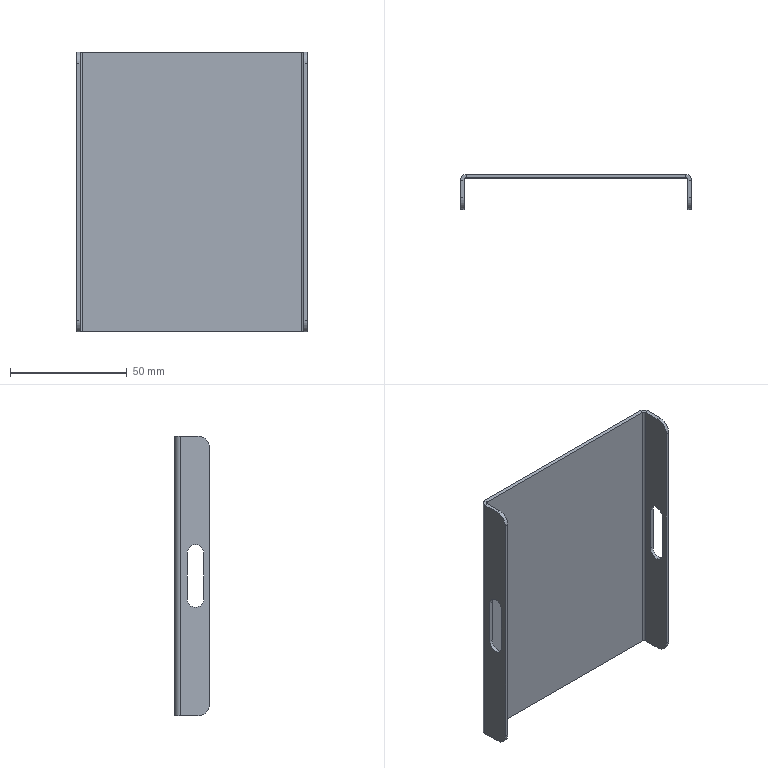Component | SolidWorks | AA-1_CoverPlate-1 | 1 solid | 36 faces | box 99 x 15 x 120 mm | volume 21842 mm3 | plane 22 | cylinder 14 | commonest cylinder face diameters 7 x6 10 x4 5 x2 2 x2
STEP:
#1=CARTESIAN_POINT('',(-19.184,-10.286,29.016));
#2=VERTEX_POINT('',#1);
#3=CARTESIAN_POINT('',(-19.184,-10.148,28.878));
#4=VERTEX_POINT('',#3);
#5=CARTESIAN_POINT('',(-19.184,-10.286,28.878));
#6=DIRECTION('',(-1.,0.,-0.));
#7=DIRECTION('',(0.,-1.,0.));
#8=AXIS2_PLACEMENT_3D('',#5,#6,#7);
#9=CIRCLE('',#8,0.1378);
#10=EDGE_CURVE('',#2,#4,#9,.T.);
#11=ORIENTED_EDGE('',*,*,#10,.F.);
#12=CARTESIAN_POINT('',(-19.243,-10.286,29.016));
#13=VERTEX_POINT('',#12);
#14=CARTESIAN_POINT('',(-15.345,-10.286,29.016));
#15=DIRECTION('',(-1.,0.,-0.));
#16=VECTOR('',#15,39.37);
#17=LINE('',#14,#16);
#18=EDGE_CURVE('',#2,#13,#17,.T.);
#19=ORIENTED_EDGE('',*,*,#18,.T.);
#20=CARTESIAN_POINT('',(-19.243,-10.148,28.878));
#21=VERTEX_POINT('',#20);
#22=CARTESIAN_POINT('',(-19.243,-10.286,28.878));
#23=DIRECTION('',(-1.,0.,-0.));
#24=DIRECTION('',(0.,0.,1.));
#25=AXIS2_PLACEMENT_3D('',#22,#23,#24);
#26=CIRCLE('',#25,0.1378);
#27=EDGE_CURVE('',#13,#21,#26,.T.);
#28=ORIENTED_EDGE('',*,*,#27,.T.);
#29=CARTESIAN_POINT('',(-15.345,-10.148,28.878));
#30=DIRECTION('',(-1.,0.,-0.));
#31=VECTOR('',#30,39.37);
#32=LINE('',#29,#31);
#33=EDGE_CURVE('',#4,#21,#32,.T.);
#34=ORIENTED_EDGE('',*,*,#33,.F.);
#35=EDGE_LOOP('',(#11,#19,#28,#34));
#36=FACE_OUTER_BOUND('',#35,.T.);
#37=CARTESIAN_POINT('',(-15.345,-10.286,28.878));
#38=DIRECTION('',(-1.,0.,-0.));
#39=DIRECTION('',(0.,0.,1.));
#40=AXIS2_PLACEMENT_3D('',#37,#38,#39);
#41=CYLINDRICAL_SURFACE('',#40,0.1378);
#42=ADVANCED_FACE('',(#36),#41,.F.);
#43=CARTESIAN_POINT('',(-15.345,-10.286,29.016));
#44=VERTEX_POINT('',#43);
#45=CARTESIAN_POINT('',(-15.345,-10.148,28.878));
#46=VERTEX_POINT('',#45);
#47=CARTESIAN_POINT('',(-15.345,-10.286,28.878));
#48=DIRECTION('',(-1.,0.,-0.));
#49=DIRECTION('',(0.,0.,1.));
#50=AXIS2_PLACEMENT_3D('',#47,#48,#49);
#51=CIRCLE('',#50,0.1378);
#52=EDGE_CURVE('',#44,#46,#51,.T.);
#53=ORIENTED_EDGE('',*,*,#52,.F.);
#54=CARTESIAN_POINT('',(-15.404,-10.286,29.016));
#55=VERTEX_POINT('',#54);
#56=CARTESIAN_POINT('',(-15.345,-10.286,29.016));
#57=DIRECTION('',(-1.,0.,-0.));
#58=VECTOR('',#57,39.37);
#59=LINE('',#56,#58);
#60=EDGE_CURVE('',#44,#55,#59,.T.);
#61=ORIENTED_EDGE('',*,*,#60,.T.);
#62=CARTESIAN_POINT('',(-15.404,-10.148,28.878));
#63=VERTEX_POINT('',#62);
#64=CARTESIAN_POINT('',(-15.404,-10.286,28.878));
#65=DIRECTION('',(-1.,-0.,-0.));
#66=DIRECTION('',(0.,-1.,0.));
#67=AXIS2_PLACEMENT_3D('',#64,#65,#66);
#68=CIRCLE('',#67,0.1378);
#69=EDGE_CURVE('',#55,#63,#68,.T.);
#70=ORIENTED_EDGE('',*,*,#69,.T.);
#71=CARTESIAN_POINT('',(-15.345,-10.148,28.878));
#72=DIRECTION('',(-1.,0.,-0.));
#73=VECTOR('',#72,39.37);
#74=LINE('',#71,#73);
#75=EDGE_CURVE('',#46,#63,#74,.T.);
#76=ORIENTED_EDGE('',*,*,#75,.F.);
#77=EDGE_LOOP('',(#53,#61,#70,#76));
#78=FACE_OUTER_BOUND('',#77,.T.);
#79=CARTESIAN_POINT('',(-15.345,-10.286,28.878));
#80=DIRECTION('',(-1.,0.,-0.));
#81=DIRECTION('',(0.,0.,1.));
#82=AXIS2_PLACEMENT_3D('',#79,#80,#81);
#83=CYLINDRICAL_SURFACE('',#82,0.1378);
#84=ADVANCED_FACE('',(#78),#83,.F.);
#85=CARTESIAN_POINT('',(-19.145,-9.932,30.846));
#86=VERTEX_POINT('',#85);
#87=CARTESIAN_POINT('',(-15.444,-9.932,30.846));
#88=VERTEX_POINT('',#87);
#89=CARTESIAN_POINT('',(-15.444,-9.932,30.846));
#90=DIRECTION('',(1.,-0.,0.));
#91=VECTOR('',#90,39.37);
#92=LINE('',#89,#91);
#93=EDGE_CURVE('',#86,#88,#92,.T.);
#94=ORIENTED_EDGE('',*,*,#93,.F.);
#95=CARTESIAN_POINT('',(-19.145,-9.991,30.846));
#96=VERTEX_POINT('',#95);
#97=CARTESIAN_POINT('',(-19.145,-9.991,30.846));
#98=DIRECTION('',(0.,1.,-0.));
#99=VECTOR('',#98,39.37);
#100=LINE('',#97,#99);
#101=EDGE_CURVE('',#96,#86,#100,.T.);
#102=ORIENTED_EDGE('',*,*,#101,.F.);
#103=CARTESIAN_POINT('',(-15.444,-9.991,30.846));
#104=VERTEX_POINT('',#103);
#105=CARTESIAN_POINT('',(-15.444,-9.991,30.846));
#106=DIRECTION('',(1.,-0.,0.));
#107=VECTOR('',#106,39.37);
#108=LINE('',#105,#107);
#109=EDGE_CURVE('',#96,#104,#108,.T.);
#110=ORIENTED_EDGE('',*,*,#109,.T.);
#111=CARTESIAN_POINT('',(-15.444,-9.991,30.846));
#112=DIRECTION('',(0.,1.,-0.));
#113=VECTOR('',#112,39.37);
#114=LINE('',#111,#113);
#115=EDGE_CURVE('',#104,#88,#114,.T.);
#116=ORIENTED_EDGE('',*,*,#115,.T.);
#117=EDGE_LOOP('',(#94,#102,#110,#116));
#118=FACE_OUTER_BOUND('',#117,.T.);
#119=CARTESIAN_POINT('',(-15.444,-9.991,30.846));
#120=DIRECTION('',(-0.,0.,1.));
#121=DIRECTION('',(1.,-0.,0.));
#122=AXIS2_PLACEMENT_3D('',#119,#120,#121);
#123=PLANE('',#122);
#124=ADVANCED_FACE('',(#118),#123,.T.);
#125=CARTESIAN_POINT('',(-15.444,-9.932,26.122));
#126=VERTEX_POINT('',#125);
#127=CARTESIAN_POINT('',(-19.145,-9.932,26.122));
#128=VERTEX_POINT('',#127);
#129=CARTESIAN_POINT('',(-15.444,-9.932,26.122));
#130=DIRECTION('',(-1.,0.,-0.));
#131=VECTOR('',#130,39.37);
#132=LINE('',#129,#131);
#133=EDGE_CURVE('',#126,#128,#132,.T.);
#134=ORIENTED_EDGE('',*,*,#133,.F.);
#135=CARTESIAN_POINT('',(-15.444,-9.991,26.122));
#136=VERTEX_POINT('',#135);
#137=CARTESIAN_POINT('',(-15.444,-9.991,26.122));
#138=DIRECTION('',(0.,1.,-0.));
#139=VECTOR('',#138,39.37);
#140=LINE('',#137,#139);
#141=EDGE_CURVE('',#136,#126,#140,.T.);
#142=ORIENTED_EDGE('',*,*,#141,.F.);
#143=CARTESIAN_POINT('',(-19.145,-9.991,26.122));
#144=VERTEX_POINT('',#143);
#145=CARTESIAN_POINT('',(-15.444,-9.991,26.122));
#146=DIRECTION('',(-1.,0.,-0.));
#147=VECTOR('',#146,39.37);
#148=LINE('',#145,#147);
#149=EDGE_CURVE('',#136,#144,#148,.T.);
#150=ORIENTED_EDGE('',*,*,#149,.T.);
#151=CARTESIAN_POINT('',(-19.145,-9.991,26.122));
#152=DIRECTION('',(0.,1.,-0.));
#153=VECTOR('',#152,39.37);
#154=LINE('',#151,#153);
#155=EDGE_CURVE('',#144,#128,#154,.T.);
#156=ORIENTED_EDGE('',*,*,#155,.T.);
#157=EDGE_LOOP('',(#134,#142,#150,#156));
#158=FACE_OUTER_BOUND('',#157,.T.);
#159=CARTESIAN_POINT('',(-15.444,-9.991,26.122));
#160=DIRECTION('',(0.,-0.,-1.));
#161=DIRECTION('',(-1.,0.,-0.));
#162=AXIS2_PLACEMENT_3D('',#159,#160,#161);
#163=PLANE('',#162);
#164=ADVANCED_FACE('',(#158),#163,.T.);
#165=ORIENTED_EDGE('',*,*,#109,.F.);
#166=CARTESIAN_POINT('',(-19.145,-9.991,26.122));
#167=DIRECTION('',(-0.,0.,1.));
#168=VECTOR('',#167,39.37);
#169=LINE('',#166,#168);
#170=EDGE_CURVE('',#144,#96,#169,.T.);
#171=ORIENTED_EDGE('',*,*,#170,.F.);
#172=ORIENTED_EDGE('',*,*,#149,.F.);
#173=CARTESIAN_POINT('',(-15.444,-9.991,26.122));
#174=DIRECTION('',(0.,-0.,-1.));
#175=VECTOR('',#174,39.37);
#176=LINE('',#173,#175);
#177=EDGE_CURVE('',#104,#136,#176,.T.);
#178=ORIENTED_EDGE('',*,*,#177,.F.);
#179=EDGE_LOOP('',(#165,#171,#172,#178));
#180=FACE_OUTER_BOUND('',#179,.T.);
#181=CARTESIAN_POINT('',(-17.294,-9.991,28.484));
#182=DIRECTION('',(0.,1.,-0.));
#183=DIRECTION('',(-1.,0.,-0.));
#184=AXIS2_PLACEMENT_3D('',#181,#182,#183);
#185=PLANE('',#184);
#186=ADVANCED_FACE('',(#180),#185,.F.);
#187=ORIENTED_EDGE('',*,*,#93,.T.);
#188=CARTESIAN_POINT('',(-15.444,-9.932,26.122));
#189=DIRECTION('',(0.,-0.,-1.));
#190=VECTOR('',#189,39.37);
#191=LINE('',#188,#190);
#192=EDGE_CURVE('',#88,#126,#191,.T.);
#193=ORIENTED_EDGE('',*,*,#192,.T.);
#194=ORIENTED_EDGE('',*,*,#133,.T.);
#195=CARTESIAN_POINT('',(-19.145,-9.932,26.122));
#196=DIRECTION('',(-0.,0.,1.));
#197=VECTOR('',#196,39.37);
#198=LINE('',#195,#197);
#199=EDGE_CURVE('',#128,#86,#198,.T.);
#200=ORIENTED_EDGE('',*,*,#199,.T.);
#201=EDGE_LOOP('',(#187,#193,#194,#200));
#202=FACE_OUTER_BOUND('',#201,.T.);
#203=CARTESIAN_POINT('',(-17.294,-9.932,28.484));
#204=DIRECTION('',(0.,1.,-0.));
#205=DIRECTION('',(-1.,0.,-0.));
#206=AXIS2_PLACEMENT_3D('',#203,#204,#205);
#207=PLANE('',#206);
#208=ADVANCED_FACE('',(#202),#207,.T.);
#209=CARTESIAN_POINT('',(-19.184,-10.03,30.846));
#210=VERTEX_POINT('',#209);
#211=CARTESIAN_POINT('',(-19.243,-10.03,30.846));
#212=VERTEX_POINT('',#211);
#213=CARTESIAN_POINT('',(-19.243,-10.03,30.846));
#214=DIRECTION('',(-1.,0.,-0.));
#215=VECTOR('',#214,39.37);
#216=LINE('',#213,#215);
#217=EDGE_CURVE('',#210,#212,#216,.T.);
#218=ORIENTED_EDGE('',*,*,#217,.F.);
#219=CARTESIAN_POINT('',(-19.145,-10.03,30.846));
#220=DIRECTION('',(-0.,0.,1.));
#221=DIRECTION('',(-1.,-0.,0.));
#222=AXIS2_PLACEMENT_3D('',#219,#220,#221);
#223=CIRCLE('',#222,0.03937);
#224=EDGE_CURVE('',#96,#210,#223,.T.);
#225=ORIENTED_EDGE('',*,*,#224,.F.);
#226=ORIENTED_EDGE('',*,*,#101,.T.);
#227=CARTESIAN_POINT('',(-19.145,-10.03,30.846));
#228=DIRECTION('',(-0.,0.,1.));
#229=DIRECTION('',(-1.,-0.,0.));
#230=AXIS2_PLACEMENT_3D('',#227,#228,#229);
#231=CIRCLE('',#230,0.09843);
#232=EDGE_CURVE('',#86,#212,#231,.T.);
#233=ORIENTED_EDGE('',*,*,#232,.T.);
#234=EDGE_LOOP('',(#218,#225,#226,#233));
#235=FACE_OUTER_BOUND('',#234,.T.);
#236=CARTESIAN_POINT('',(-19.145,-10.03,30.846));
#237=DIRECTION('',(-0.,0.,1.));
#238=DIRECTION('',(1.,-0.,0.));
#239=AXIS2_PLACEMENT_3D('',#236,#237,#238);
#240=PLANE('',#239);
#241=ADVANCED_FACE('',(#235),#240,.T.);
#242=CARTESIAN_POINT('',(-19.184,-10.03,26.122));
#243=VERTEX_POINT('',#242);
#244=CARTESIAN_POINT('',(-19.145,-10.03,26.122));
#245=DIRECTION('',(0.,-0.,-1.));
#246=DIRECTION('',(-1.,0.,0.));
#247=AXIS2_PLACEMENT_3D('',#244,#245,#246);
#248=CIRCLE('',#247,0.03937);
#249=EDGE_CURVE('',#243,#144,#248,.T.);
#250=ORIENTED_EDGE('',*,*,#249,.F.);
#251=CARTESIAN_POINT('',(-19.243,-10.03,26.122));
#252=VERTEX_POINT('',#251);
#253=CARTESIAN_POINT('',(-19.184,-10.03,26.122));
#254=DIRECTION('',(-1.,0.,-0.));
#255=VECTOR('',#254,39.37);
#256=LINE('',#253,#255);
#257=EDGE_CURVE('',#243,#252,#256,.T.);
#258=ORIENTED_EDGE('',*,*,#257,.T.);
#259=CARTESIAN_POINT('',(-19.145,-10.03,26.122));
#260=DIRECTION('',(0.,-0.,-1.));
#261=DIRECTION('',(-1.,0.,0.));
#262=AXIS2_PLACEMENT_3D('',#259,#260,#261);
#263=CIRCLE('',#262,0.09843);
#264=EDGE_CURVE('',#252,#128,#263,.T.);
#265=ORIENTED_EDGE('',*,*,#264,.T.);
#266=ORIENTED_EDGE('',*,*,#155,.F.);
#267=EDGE_LOOP('',(#250,#258,#265,#266));
#268=FACE_OUTER_BOUND('',#267,.T.);
#269=CARTESIAN_POINT('',(-19.145,-10.03,26.122));
#270=DIRECTION('',(-0.,0.,1.));
#271=DIRECTION('',(1.,-0.,0.));
#272=AXIS2_PLACEMENT_3D('',#269,#270,#271);
#273=PLANE('',#272);
#274=ADVANCED_FACE('',(#268),#273,.F.);
#275=ORIENTED_EDGE('',*,*,#199,.F.);
#276=ORIENTED_EDGE('',*,*,#264,.F.);
#277=CARTESIAN_POINT('',(-19.243,-10.03,28.484));
#278=DIRECTION('',(0.,-0.,-1.));
#279=VECTOR('',#278,39.37);
#280=LINE('',#277,#279);
#281=EDGE_CURVE('',#212,#252,#280,.T.);
#282=ORIENTED_EDGE('',*,*,#281,.F.);
#283=ORIENTED_EDGE('',*,*,#232,.F.);
#284=EDGE_LOOP('',(#275,#276,#282,#283));
#285=FACE_OUTER_BOUND('',#284,.T.);
#286=CARTESIAN_POINT('',(-19.145,-10.03,26.122));
#287=DIRECTION('',(0.,-0.,-1.));
#288=DIRECTION('',(-1.,0.,0.));
#289=AXIS2_PLACEMENT_3D('',#286,#287,#288);
#290=CYLINDRICAL_SURFACE('',#289,0.09843);
#291=ADVANCED_FACE('',(#285),#290,.T.);
#292=ORIENTED_EDGE('',*,*,#170,.T.);
#293=ORIENTED_EDGE('',*,*,#224,.T.);
#294=CARTESIAN_POINT('',(-19.184,-10.03,30.846));
#295=DIRECTION('',(0.,-0.,-1.));
#296=VECTOR('',#295,39.37);
#297=LINE('',#294,#296);
#298=EDGE_CURVE('',#210,#243,#297,.T.);
#299=ORIENTED_EDGE('',*,*,#298,.T.);
#300=ORIENTED_EDGE('',*,*,#249,.T.);
#301=EDGE_LOOP('',(#292,#293,#299,#300));
#302=FACE_OUTER_BOUND('',#301,.T.);
#303=CARTESIAN_POINT('',(-19.145,-10.03,26.122));
#304=DIRECTION('',(0.,-0.,-1.));
#305=DIRECTION('',(-1.,0.,0.));
#306=AXIS2_PLACEMENT_3D('',#303,#304,#305);
#307=CYLINDRICAL_SURFACE('',#306,0.03937);
#308=ADVANCED_FACE('',(#302),#307,.F.);
#309=CARTESIAN_POINT('',(-19.184,-10.325,26.122));
#310=VERTEX_POINT('',#309);
#311=CARTESIAN_POINT('',(-19.184,-9.932,26.122));
#312=DIRECTION('',(0.,1.,-0.));
#313=VECTOR('',#312,39.37);
#314=LINE('',#311,#313);
#315=EDGE_CURVE('',#310,#243,#314,.T.);
#316=ORIENTED_EDGE('',*,*,#315,.F.);
#317=CARTESIAN_POINT('',(-19.243,-10.325,26.122));
#318=VERTEX_POINT('',#317);
#319=CARTESIAN_POINT('',(-19.243,-10.325,26.122));
#320=DIRECTION('',(-1.,0.,-0.));
#321=VECTOR('',#320,39.37);
#322=LINE('',#319,#321);
#323=EDGE_CURVE('',#310,#318,#322,.T.);
#324=ORIENTED_EDGE('',*,*,#323,.T.);
#325=CARTESIAN_POINT('',(-19.243,-9.991,26.122));
#326=DIRECTION('',(0.,1.,-0.));
#327=VECTOR('',#326,39.37);
#328=LINE('',#325,#327);
#329=EDGE_CURVE('',#318,#252,#328,.T.);
#330=ORIENTED_EDGE('',*,*,#329,.T.);
#331=ORIENTED_EDGE('',*,*,#257,.F.);
#332=EDGE_LOOP('',(#316,#324,#330,#331));
#333=FACE_OUTER_BOUND('',#332,.T.);
#334=CARTESIAN_POINT('',(-19.243,-9.991,26.122));
#335=DIRECTION('',(0.,-0.,-1.));
#336=DIRECTION('',(-1.,0.,-0.));
#337=AXIS2_PLACEMENT_3D('',#334,#335,#336);
#338=PLANE('',#337);
#339=ADVANCED_FACE('',(#333),#338,.T.);
#340=CARTESIAN_POINT('',(-19.243,-10.325,30.846));
#341=VERTEX_POINT('',#340);
#342=CARTESIAN_POINT('',(-19.243,-10.522,30.846));
#343=DIRECTION('',(-0.,-1.,0.));
#344=VECTOR('',#343,39.37);
#345=LINE('',#342,#344);
#346=EDGE_CURVE('',#212,#341,#345,.T.);
#347=ORIENTED_EDGE('',*,*,#346,.T.);
#348=CARTESIAN_POINT('',(-19.184,-10.325,30.846));
#349=VERTEX_POINT('',#348);
#350=CARTESIAN_POINT('',(-19.243,-10.325,30.846));
#351=DIRECTION('',(1.,-0.,0.));
#352=VECTOR('',#351,39.37);
#353=LINE('',#350,#352);
#354=EDGE_CURVE('',#341,#349,#353,.T.);
#355=ORIENTED_EDGE('',*,*,#354,.T.);
#356=CARTESIAN_POINT('',(-19.184,-9.932,30.846));
#357=DIRECTION('',(-0.,-1.,0.));
#358=VECTOR('',#357,39.37);
#359=LINE('',#356,#358);
#360=EDGE_CURVE('',#210,#349,#359,.T.);
#361=ORIENTED_EDGE('',*,*,#360,.F.);
#362=ORIENTED_EDGE('',*,*,#217,.T.);
#363=EDGE_LOOP('',(#347,#355,#361,#362));
#364=FACE_OUTER_BOUND('',#363,.T.);
#365=CARTESIAN_POINT('',(-19.243,-10.522,30.846));
#366=DIRECTION('',(-0.,0.,1.));
#367=DIRECTION('',(1.,-0.,0.));
#368=AXIS2_PLACEMENT_3D('',#365,#366,#367);
#369=PLANE('',#368);
#370=ADVANCED_FACE('',(#364),#369,.T.);
#371=CARTESIAN_POINT('',(-19.243,-10.148,28.091));
#372=VERTEX_POINT('',#371);
#373=CARTESIAN_POINT('',(-19.243,-10.424,28.091));
#374=VERTEX_POINT('',#373);
#375=CARTESIAN_POINT('',(-19.243,-10.286,28.091));
#376=DIRECTION('',(-1.,0.,-0.));
#377=DIRECTION('',(0.,0.,1.));
#378=AXIS2_PLACEMENT_3D('',#375,#376,#377);
#379=CIRCLE('',#378,0.1378);
#380=EDGE_CURVE('',#372,#374,#379,.T.);
#381=ORIENTED_EDGE('',*,*,#380,.F.);
#382=CARTESIAN_POINT('',(-19.243,-10.148,28.091));
#383=DIRECTION('',(0.,-0.,-1.));
#384=VECTOR('',#383,39.37);
#385=LINE('',#382,#384);
#386=EDGE_CURVE('',#21,#372,#385,.T.);
#387=ORIENTED_EDGE('',*,*,#386,.F.);
#388=ORIENTED_EDGE('',*,*,#27,.F.);
#389=CARTESIAN_POINT('',(-19.243,-10.424,28.878));
#390=VERTEX_POINT('',#389);
#391=CARTESIAN_POINT('',(-19.243,-10.286,28.878));
#392=DIRECTION('',(-1.,0.,-0.));
#393=DIRECTION('',(0.,0.,1.));
#394=AXIS2_PLACEMENT_3D('',#391,#392,#393);
#395=CIRCLE('',#394,0.1378);
#396=EDGE_CURVE('',#390,#13,#395,.T.);
#397=ORIENTED_EDGE('',*,*,#396,.F.);
#398=CARTESIAN_POINT('',(-19.243,-10.424,28.091));
#399=DIRECTION('',(-0.,0.,1.));
#400=VECTOR('',#399,39.37);
#401=LINE('',#398,#400);
#402=EDGE_CURVE('',#374,#390,#401,.T.);
#403=ORIENTED_EDGE('',*,*,#402,.F.);
#404=EDGE_LOOP('',(#381,#387,#388,#397,#403));
#405=FACE_BOUND('',#404,.T.);
#406=CARTESIAN_POINT('',(-19.243,-10.522,30.65));
#407=VERTEX_POINT('',#406);
#408=CARTESIAN_POINT('',(-19.243,-10.522,26.319));
#409=VERTEX_POINT('',#408);
#410=CARTESIAN_POINT('',(-19.243,-10.522,26.122));
#411=DIRECTION('',(0.,-0.,-1.));
#412=VECTOR('',#411,39.37);
#413=LINE('',#410,#412);
#414=EDGE_CURVE('',#407,#409,#413,.T.);
#415=ORIENTED_EDGE('',*,*,#414,.F.);
#416=CARTESIAN_POINT('',(-19.243,-10.325,30.65));
#417=DIRECTION('',(-1.,0.,-0.));
#418=DIRECTION('',(0.,-1.,0.));
#419=AXIS2_PLACEMENT_3D('',#416,#417,#418);
#420=CIRCLE('',#419,0.1969);
#421=EDGE_CURVE('',#407,#341,#420,.T.);
#422=ORIENTED_EDGE('',*,*,#421,.T.);
#423=ORIENTED_EDGE('',*,*,#346,.F.);
#424=ORIENTED_EDGE('',*,*,#281,.T.);
#425=ORIENTED_EDGE('',*,*,#329,.F.);
#426=CARTESIAN_POINT('',(-19.243,-10.325,26.319));
#427=DIRECTION('',(-1.,0.,-0.));
#428=DIRECTION('',(0.,-1.,0.));
#429=AXIS2_PLACEMENT_3D('',#426,#427,#428);
#430=CIRCLE('',#429,0.1969);
#431=EDGE_CURVE('',#318,#409,#430,.T.);
#432=ORIENTED_EDGE('',*,*,#431,.T.);
#433=EDGE_LOOP('',(#415,#422,#423,#424,#425,#432));
#434=FACE_OUTER_BOUND('',#433,.T.);
#435=CARTESIAN_POINT('',(-19.243,-9.932,28.484));
#436=DIRECTION('',(-1.,0.,-0.));
#437=DIRECTION('',(-0.,-1.,0.));
#438=AXIS2_PLACEMENT_3D('',#435,#436,#437);
#439=PLANE('',#438);
#440=ADVANCED_FACE('',(#405,#434),#439,.T.);
#441=CARTESIAN_POINT('',(-19.184,-10.148,28.091));
#442=VERTEX_POINT('',#441);
#443=CARTESIAN_POINT('',(-19.184,-10.148,28.484));
#444=DIRECTION('',(0.,-0.,-1.));
#445=VECTOR('',#444,39.37);
#446=LINE('',#443,#445);
#447=EDGE_CURVE('',#4,#442,#446,.T.);
#448=ORIENTED_EDGE('',*,*,#447,.T.);
#449=CARTESIAN_POINT('',(-19.184,-10.424,28.091));
#450=VERTEX_POINT('',#449);
#451=CARTESIAN_POINT('',(-19.184,-10.286,28.091));
#452=DIRECTION('',(-1.,0.,-0.));
#453=DIRECTION('',(0.,-1.,0.));
#454=AXIS2_PLACEMENT_3D('',#451,#452,#453);
#455=CIRCLE('',#454,0.1378);
#456=EDGE_CURVE('',#442,#450,#455,.T.);
#457=ORIENTED_EDGE('',*,*,#456,.T.);
#458=CARTESIAN_POINT('',(-19.184,-10.424,28.878));
#459=VERTEX_POINT('',#458);
#460=CARTESIAN_POINT('',(-19.184,-10.424,28.484));
#461=DIRECTION('',(-0.,0.,1.));
#462=VECTOR('',#461,39.37);
#463=LINE('',#460,#462);
#464=EDGE_CURVE('',#450,#459,#463,.T.);
#465=ORIENTED_EDGE('',*,*,#464,.T.);
#466=CARTESIAN_POINT('',(-19.184,-10.286,28.878));
#467=DIRECTION('',(-1.,0.,-0.));
#468=DIRECTION('',(0.,-1.,0.));
#469=AXIS2_PLACEMENT_3D('',#466,#467,#468);
#470=CIRCLE('',#469,0.1378);
#471=EDGE_CURVE('',#459,#2,#470,.T.);
#472=ORIENTED_EDGE('',*,*,#471,.T.);
#473=ORIENTED_EDGE('',*,*,#10,.T.);
#474=EDGE_LOOP('',(#448,#457,#465,#472,#473));
#475=FACE_BOUND('',#474,.T.);
#476=ORIENTED_EDGE('',*,*,#360,.T.);
#477=CARTESIAN_POINT('',(-19.184,-10.522,30.65));
#478=VERTEX_POINT('',#477);
#479=CARTESIAN_POINT('',(-19.184,-10.325,30.65));
#480=DIRECTION('',(1.,-0.,0.));
#481=DIRECTION('',(0.,-1.,0.));
#482=AXIS2_PLACEMENT_3D('',#479,#480,#481);
#483=CIRCLE('',#482,0.1969);
#484=EDGE_CURVE('',#349,#478,#483,.T.);
#485=ORIENTED_EDGE('',*,*,#484,.T.);
#486=CARTESIAN_POINT('',(-19.184,-10.522,26.319));
#487=VERTEX_POINT('',#486);
#488=CARTESIAN_POINT('',(-19.184,-10.522,28.484));
#489=DIRECTION('',(0.,-0.,-1.));
#490=VECTOR('',#489,39.37);
#491=LINE('',#488,#490);
#492=EDGE_CURVE('',#478,#487,#491,.T.);
#493=ORIENTED_EDGE('',*,*,#492,.T.);
#494=CARTESIAN_POINT('',(-19.184,-10.325,26.319));
#495=DIRECTION('',(1.,-0.,0.));
#496=DIRECTION('',(0.,-1.,0.));
#497=AXIS2_PLACEMENT_3D('',#494,#495,#496);
#498=CIRCLE('',#497,0.1969);
#499=EDGE_CURVE('',#487,#310,#498,.T.);
#500=ORIENTED_EDGE('',*,*,#499,.T.);
#501=ORIENTED_EDGE('',*,*,#315,.T.);
#502=ORIENTED_EDGE('',*,*,#298,.F.);
#503=EDGE_LOOP('',(#476,#485,#493,#500,#501,#502));
#504=FACE_OUTER_BOUND('',#503,.T.);
#505=CARTESIAN_POINT('',(-19.184,-9.932,28.484));
#506=DIRECTION('',(-1.,0.,-0.));
#507=DIRECTION('',(-0.,-1.,0.));
#508=AXIS2_PLACEMENT_3D('',#505,#506,#507);
#509=PLANE('',#508);
#510=ADVANCED_FACE('',(#475,#504),#509,.F.);
#511=ORIENTED_EDGE('',*,*,#492,.F.);
#512=CARTESIAN_POINT('',(-19.243,-10.522,30.65));
#513=DIRECTION('',(-1.,0.,-0.));
#514=VECTOR('',#513,39.37);
#515=LINE('',#512,#514);
#516=EDGE_CURVE('',#478,#407,#515,.T.);
#517=ORIENTED_EDGE('',*,*,#516,.T.);
#518=ORIENTED_EDGE('',*,*,#414,.T.);
#519=CARTESIAN_POINT('',(-19.243,-10.522,26.319));
#520=DIRECTION('',(1.,-0.,0.));
#521=VECTOR('',#520,39.37);
#522=LINE('',#519,#521);
#523=EDGE_CURVE('',#409,#487,#522,.T.);
#524=ORIENTED_EDGE('',*,*,#523,.T.);
#525=EDGE_LOOP('',(#511,#517,#518,#524));
#526=FACE_OUTER_BOUND('',#525,.T.);
#527=CARTESIAN_POINT('',(-19.243,-10.522,26.122));
#528=DIRECTION('',(-0.,-1.,0.));
#529=DIRECTION('',(1.,-0.,0.));
#530=AXIS2_PLACEMENT_3D('',#527,#528,#529);
#531=PLANE('',#530);
#532=ADVANCED_FACE('',(#526),#531,.T.);
#533=CARTESIAN_POINT('',(-15.404,-10.03,26.122));
#534=VERTEX_POINT('',#533);
#535=CARTESIAN_POINT('',(-15.345,-10.03,26.122));
#536=VERTEX_POINT('',#535);
#537=CARTESIAN_POINT('',(-15.345,-10.03,26.122));
#538=DIRECTION('',(1.,0.,0.));
#539=VECTOR('',#538,39.37);
#540=LINE('',#537,#539);
#541=EDGE_CURVE('',#534,#536,#540,.T.);
#542=ORIENTED_EDGE('',*,*,#541,.F.);
#543=CARTESIAN_POINT('',(-15.444,-10.03,26.122));
#544=DIRECTION('',(0.,-0.,-1.));
#545=DIRECTION('',(1.,0.,0.));
#546=AXIS2_PLACEMENT_3D('',#543,#544,#545);
#547=CIRCLE('',#546,0.03937);
#548=EDGE_CURVE('',#136,#534,#547,.T.);
#549=ORIENTED_EDGE('',*,*,#548,.F.);
#550=ORIENTED_EDGE('',*,*,#141,.T.);
#551=CARTESIAN_POINT('',(-15.444,-10.03,26.122));
#552=DIRECTION('',(0.,-0.,-1.));
#553=DIRECTION('',(1.,0.,0.));
#554=AXIS2_PLACEMENT_3D('',#551,#552,#553);
#555=CIRCLE('',#554,0.09843);
#556=EDGE_CURVE('',#126,#536,#555,.T.);
#557=ORIENTED_EDGE('',*,*,#556,.T.);
#558=EDGE_LOOP('',(#542,#549,#550,#557));
#559=FACE_OUTER_BOUND('',#558,.T.);
#560=CARTESIAN_POINT('',(-15.444,-10.03,26.122));
#561=DIRECTION('',(0.,-0.,-1.));
#562=DIRECTION('',(-1.,0.,-0.));
#563=AXIS2_PLACEMENT_3D('',#560,#561,#562);
#564=PLANE('',#563);
#565=ADVANCED_FACE('',(#559),#564,.T.);
#566=CARTESIAN_POINT('',(-15.404,-10.03,30.846));
#567=VERTEX_POINT('',#566);
#568=CARTESIAN_POINT('',(-15.444,-10.03,30.846));
#569=DIRECTION('',(-0.,0.,1.));
#570=DIRECTION('',(1.,0.,0.));
#571=AXIS2_PLACEMENT_3D('',#568,#569,#570);
#572=CIRCLE('',#571,0.03937);
#573=EDGE_CURVE('',#567,#104,#572,.T.);
#574=ORIENTED_EDGE('',*,*,#573,.F.);
#575=CARTESIAN_POINT('',(-15.345,-10.03,30.846));
#576=VERTEX_POINT('',#575);
#577=CARTESIAN_POINT('',(-15.404,-10.03,30.846));
#578=DIRECTION('',(1.,0.,0.));
#579=VECTOR('',#578,39.37);
#580=LINE('',#577,#579);
#581=EDGE_CURVE('',#567,#576,#580,.T.);
#582=ORIENTED_EDGE('',*,*,#581,.T.);
#583=CARTESIAN_POINT('',(-15.444,-10.03,30.846));
#584=DIRECTION('',(-0.,0.,1.));
#585=DIRECTION('',(1.,0.,0.));
#586=AXIS2_PLACEMENT_3D('',#583,#584,#585);
#587=CIRCLE('',#586,0.09843);
#588=EDGE_CURVE('',#576,#88,#587,.T.);
#589=ORIENTED_EDGE('',*,*,#588,.T.);
#590=ORIENTED_EDGE('',*,*,#115,.F.);
#591=EDGE_LOOP('',(#574,#582,#589,#590));
#592=FACE_OUTER_BOUND('',#591,.T.);
#593=CARTESIAN_POINT('',(-15.444,-10.03,30.846));
#594=DIRECTION('',(0.,-0.,-1.));
#595=DIRECTION('',(-1.,0.,-0.));
#596=AXIS2_PLACEMENT_3D('',#593,#594,#595);
#597=PLANE('',#596);
#598=ADVANCED_FACE('',(#592),#597,.F.);
#599=ORIENTED_EDGE('',*,*,#192,.F.);
#600=ORIENTED_EDGE('',*,*,#588,.F.);
#601=CARTESIAN_POINT('',(-15.345,-10.03,26.122));
#602=DIRECTION('',(0.,-0.,-1.));
#603=VECTOR('',#602,39.37);
#604=LINE('',#601,#603);
#605=EDGE_CURVE('',#576,#536,#604,.T.);
#606=ORIENTED_EDGE('',*,*,#605,.T.);
#607=ORIENTED_EDGE('',*,*,#556,.F.);
#608=EDGE_LOOP('',(#599,#600,#606,#607));
#609=FACE_OUTER_BOUND('',#608,.T.);
#610=CARTESIAN_POINT('',(-15.444,-10.03,30.846));
#611=DIRECTION('',(-0.,0.,1.));
#612=DIRECTION('',(1.,0.,0.));
#613=AXIS2_PLACEMENT_3D('',#610,#611,#612);
#614=CYLINDRICAL_SURFACE('',#613,0.09843);
#615=ADVANCED_FACE('',(#609),#614,.T.);
#616=ORIENTED_EDGE('',*,*,#177,.T.);
#617=ORIENTED_EDGE('',*,*,#548,.T.);
#618=CARTESIAN_POINT('',(-15.404,-10.03,26.122));
#619=DIRECTION('',(-0.,0.,1.));
#620=VECTOR('',#619,39.37);
#621=LINE('',#618,#620);
#622=EDGE_CURVE('',#534,#567,#621,.T.);
#623=ORIENTED_EDGE('',*,*,#622,.T.);
#624=ORIENTED_EDGE('',*,*,#573,.T.);
#625=EDGE_LOOP('',(#616,#617,#623,#624));
#626=FACE_OUTER_BOUND('',#625,.T.);
#627=CARTESIAN_POINT('',(-15.444,-10.03,30.846));
#628=DIRECTION('',(-0.,0.,1.));
#629=DIRECTION('',(1.,0.,0.));
#630=AXIS2_PLACEMENT_3D('',#627,#628,#629);
#631=CYLINDRICAL_SURFACE('',#630,0.03937);
#632=ADVANCED_FACE('',(#626),#631,.F.);
#633=CARTESIAN_POINT('',(-15.345,-10.325,26.122));
#634=VERTEX_POINT('',#633);
#635=CARTESIAN_POINT('',(-15.345,-9.991,26.122));
#636=DIRECTION('',(0.,-1.,0.));
#637=VECTOR('',#636,39.37);
#638=LINE('',#635,#637);
#639=EDGE_CURVE('',#536,#634,#638,.T.);
#640=ORIENTED_EDGE('',*,*,#639,.T.);
#641=CARTESIAN_POINT('',(-15.404,-10.325,26.122));
#642=VERTEX_POINT('',#641);
#643=CARTESIAN_POINT('',(-15.345,-10.325,26.122));
#644=DIRECTION('',(-1.,-0.,-0.));
#645=VECTOR('',#644,39.37);
#646=LINE('',#643,#645);
#647=EDGE_CURVE('',#634,#642,#646,.T.);
#648=ORIENTED_EDGE('',*,*,#647,.T.);
#649=CARTESIAN_POINT('',(-15.404,-9.932,26.122));
#650=DIRECTION('',(0.,-1.,0.));
#651=VECTOR('',#650,39.37);
#652=LINE('',#649,#651);
#653=EDGE_CURVE('',#534,#642,#652,.T.);
#654=ORIENTED_EDGE('',*,*,#653,.F.);
#655=ORIENTED_EDGE('',*,*,#541,.T.);
#656=EDGE_LOOP('',(#640,#648,#654,#655));
#657=FACE_OUTER_BOUND('',#656,.T.);
#658=CARTESIAN_POINT('',(-15.345,-9.991,26.122));
#659=DIRECTION('',(0.,-0.,-1.));
#660=DIRECTION('',(-1.,0.,-0.));
#661=AXIS2_PLACEMENT_3D('',#658,#659,#660);
#662=PLANE('',#661);
#663=ADVANCED_FACE('',(#657),#662,.T.);
#664=CARTESIAN_POINT('',(-15.404,-10.325,30.846));
#665=VERTEX_POINT('',#664);
#666=CARTESIAN_POINT('',(-15.404,-9.932,30.846));
#667=DIRECTION('',(-0.,1.,-0.));
#668=VECTOR('',#667,39.37);
#669=LINE('',#666,#668);
#670=EDGE_CURVE('',#665,#567,#669,.T.);
#671=ORIENTED_EDGE('',*,*,#670,.F.);
#672=CARTESIAN_POINT('',(-15.345,-10.325,30.846));
#673=VERTEX_POINT('',#672);
#674=CARTESIAN_POINT('',(-15.345,-10.325,30.846));
#675=DIRECTION('',(1.,0.,0.));
#676=VECTOR('',#675,39.37);
#677=LINE('',#674,#676);
#678=EDGE_CURVE('',#665,#673,#677,.T.);
#679=ORIENTED_EDGE('',*,*,#678,.T.);
#680=CARTESIAN_POINT('',(-15.345,-10.522,30.846));
#681=DIRECTION('',(-0.,1.,-0.));
#682=VECTOR('',#681,39.37);
#683=LINE('',#680,#682);
#684=EDGE_CURVE('',#673,#576,#683,.T.);
#685=ORIENTED_EDGE('',*,*,#684,.T.);
#686=ORIENTED_EDGE('',*,*,#581,.F.);
#687=EDGE_LOOP('',(#671,#679,#685,#686));
#688=FACE_OUTER_BOUND('',#687,.T.);
#689=CARTESIAN_POINT('',(-15.345,-10.522,30.846));
#690=DIRECTION('',(-0.,0.,1.));
#691=DIRECTION('',(1.,-0.,0.));
#692=AXIS2_PLACEMENT_3D('',#689,#690,#691);
#693=PLANE('',#692);
#694=ADVANCED_FACE('',(#688),#693,.T.);
#695=CARTESIAN_POINT('',(-15.345,-10.148,28.091));
#696=VERTEX_POINT('',#695);
#697=CARTESIAN_POINT('',(-15.345,-10.148,28.091));
#698=DIRECTION('',(0.,-0.,-1.));
#699=VECTOR('',#698,39.37);
#700=LINE('',#697,#699);
#701=EDGE_CURVE('',#46,#696,#700,.T.);
#702=ORIENTED_EDGE('',*,*,#701,.T.);
#703=CARTESIAN_POINT('',(-15.345,-10.424,28.091));
#704=VERTEX_POINT('',#703);
#705=CARTESIAN_POINT('',(-15.345,-10.286,28.091));
#706=DIRECTION('',(-1.,0.,-0.));
#707=DIRECTION('',(0.,0.,1.));
#708=AXIS2_PLACEMENT_3D('',#705,#706,#707);
#709=CIRCLE('',#708,0.1378);
#710=EDGE_CURVE('',#696,#704,#709,.T.);
#711=ORIENTED_EDGE('',*,*,#710,.T.);
#712=CARTESIAN_POINT('',(-15.345,-10.424,28.878));
#713=VERTEX_POINT('',#712);
#714=CARTESIAN_POINT('',(-15.345,-10.424,28.091));
#715=DIRECTION('',(-0.,0.,1.));
#716=VECTOR('',#715,39.37);
#717=LINE('',#714,#716);
#718=EDGE_CURVE('',#704,#713,#717,.T.);
#719=ORIENTED_EDGE('',*,*,#718,.T.);
#720=CARTESIAN_POINT('',(-15.345,-10.286,28.878));
#721=DIRECTION('',(-1.,0.,-0.));
#722=DIRECTION('',(0.,0.,1.));
#723=AXIS2_PLACEMENT_3D('',#720,#721,#722);
#724=CIRCLE('',#723,0.1378);
#725=EDGE_CURVE('',#713,#44,#724,.T.);
#726=ORIENTED_EDGE('',*,*,#725,.T.);
#727=ORIENTED_EDGE('',*,*,#52,.T.);
#728=EDGE_LOOP('',(#702,#711,#719,#726,#727));
#729=FACE_BOUND('',#728,.T.);
#730=ORIENTED_EDGE('',*,*,#684,.F.);
#731=CARTESIAN_POINT('',(-15.345,-10.522,30.65));
#732=VERTEX_POINT('',#731);
#733=CARTESIAN_POINT('',(-15.345,-10.325,30.65));
#734=DIRECTION('',(1.,0.,0.));
#735=DIRECTION('',(0.,-1.,0.));
#736=AXIS2_PLACEMENT_3D('',#733,#734,#735);
#737=CIRCLE('',#736,0.1969);
#738=EDGE_CURVE('',#673,#732,#737,.T.);
#739=ORIENTED_EDGE('',*,*,#738,.T.);
#740=CARTESIAN_POINT('',(-15.345,-10.522,26.319));
#741=VERTEX_POINT('',#740);
#742=CARTESIAN_POINT('',(-15.345,-10.522,26.122));
#743=DIRECTION('',(-0.,0.,1.));
#744=VECTOR('',#743,39.37);
#745=LINE('',#742,#744);
#746=EDGE_CURVE('',#741,#732,#745,.T.);
#747=ORIENTED_EDGE('',*,*,#746,.F.);
#748=CARTESIAN_POINT('',(-15.345,-10.325,26.319));
#749=DIRECTION('',(1.,0.,0.));
#750=DIRECTION('',(0.,-1.,0.));
#751=AXIS2_PLACEMENT_3D('',#748,#749,#750);
#752=CIRCLE('',#751,0.1969);
#753=EDGE_CURVE('',#741,#634,#752,.T.);
#754=ORIENTED_EDGE('',*,*,#753,.T.);
#755=ORIENTED_EDGE('',*,*,#639,.F.);
#756=ORIENTED_EDGE('',*,*,#605,.F.);
#757=EDGE_LOOP('',(#730,#739,#747,#754,#755,#756));
#758=FACE_OUTER_BOUND('',#757,.T.);
#759=CARTESIAN_POINT('',(-15.345,-9.932,28.484));
#760=DIRECTION('',(-1.,-0.,-0.));
#761=DIRECTION('',(0.,-1.,0.));
#762=AXIS2_PLACEMENT_3D('',#759,#760,#761);
#763=PLANE('',#762);
#764=ADVANCED_FACE('',(#729,#758),#763,.F.);
#765=CARTESIAN_POINT('',(-15.404,-10.148,28.091));
#766=VERTEX_POINT('',#765);
#767=CARTESIAN_POINT('',(-15.404,-10.424,28.091));
#768=VERTEX_POINT('',#767);
#769=CARTESIAN_POINT('',(-15.404,-10.286,28.091));
#770=DIRECTION('',(-1.,-0.,-0.));
#771=DIRECTION('',(0.,-1.,0.));
#772=AXIS2_PLACEMENT_3D('',#769,#770,#771);
#773=CIRCLE('',#772,0.1378);
#774=EDGE_CURVE('',#766,#768,#773,.T.);
#775=ORIENTED_EDGE('',*,*,#774,.F.);
#776=CARTESIAN_POINT('',(-15.404,-10.148,28.484));
#777=DIRECTION('',(0.,-0.,-1.));
#778=VECTOR('',#777,39.37);
#779=LINE('',#776,#778);
#780=EDGE_CURVE('',#63,#766,#779,.T.);
#781=ORIENTED_EDGE('',*,*,#780,.F.);
#782=ORIENTED_EDGE('',*,*,#69,.F.);
#783=CARTESIAN_POINT('',(-15.404,-10.424,28.878));
#784=VERTEX_POINT('',#783);
#785=CARTESIAN_POINT('',(-15.404,-10.286,28.878));
#786=DIRECTION('',(-1.,-0.,-0.));
#787=DIRECTION('',(0.,-1.,0.));
#788=AXIS2_PLACEMENT_3D('',#785,#786,#787);
#789=CIRCLE('',#788,0.1378);
#790=EDGE_CURVE('',#784,#55,#789,.T.);
#791=ORIENTED_EDGE('',*,*,#790,.F.);
#792=CARTESIAN_POINT('',(-15.404,-10.424,28.484));
#793=DIRECTION('',(-0.,0.,1.));
#794=VECTOR('',#793,39.37);
#795=LINE('',#792,#794);
#796=EDGE_CURVE('',#768,#784,#795,.T.);
#797=ORIENTED_EDGE('',*,*,#796,.F.);
#798=EDGE_LOOP('',(#775,#781,#782,#791,#797));
#799=FACE_BOUND('',#798,.T.);
#800=CARTESIAN_POINT('',(-15.404,-10.522,26.319));
#801=VERTEX_POINT('',#800);
#802=CARTESIAN_POINT('',(-15.404,-10.522,30.65));
#803=VERTEX_POINT('',#802);
#804=CARTESIAN_POINT('',(-15.404,-10.522,28.484));
#805=DIRECTION('',(-0.,0.,1.));
#806=VECTOR('',#805,39.37);
#807=LINE('',#804,#806);
#808=EDGE_CURVE('',#801,#803,#807,.T.);
#809=ORIENTED_EDGE('',*,*,#808,.T.);
#810=CARTESIAN_POINT('',(-15.404,-10.325,30.65));
#811=DIRECTION('',(-1.,-0.,-0.));
#812=DIRECTION('',(0.,-1.,0.));
#813=AXIS2_PLACEMENT_3D('',#810,#811,#812);
#814=CIRCLE('',#813,0.1969);
#815=EDGE_CURVE('',#803,#665,#814,.T.);
#816=ORIENTED_EDGE('',*,*,#815,.T.);
#817=ORIENTED_EDGE('',*,*,#670,.T.);
#818=ORIENTED_EDGE('',*,*,#622,.F.);
#819=ORIENTED_EDGE('',*,*,#653,.T.);
#820=CARTESIAN_POINT('',(-15.404,-10.325,26.319));
#821=DIRECTION('',(-1.,-0.,-0.));
#822=DIRECTION('',(0.,-1.,0.));
#823=AXIS2_PLACEMENT_3D('',#820,#821,#822);
#824=CIRCLE('',#823,0.1969);
#825=EDGE_CURVE('',#642,#801,#824,.T.);
#826=ORIENTED_EDGE('',*,*,#825,.T.);
#827=EDGE_LOOP('',(#809,#816,#817,#818,#819,#826));
#828=FACE_OUTER_BOUND('',#827,.T.);
#829=CARTESIAN_POINT('',(-15.404,-9.932,28.484));
#830=DIRECTION('',(-1.,-0.,-0.));
#831=DIRECTION('',(0.,-1.,0.));
#832=AXIS2_PLACEMENT_3D('',#829,#830,#831);
#833=PLANE('',#832);
#834=ADVANCED_FACE('',(#799,#828),#833,.T.);
#835=ORIENTED_EDGE('',*,*,#746,.T.);
#836=CARTESIAN_POINT('',(-15.345,-10.522,30.65));
#837=DIRECTION('',(-1.,-0.,-0.));
#838=VECTOR('',#837,39.37);
#839=LINE('',#836,#838);
#840=EDGE_CURVE('',#732,#803,#839,.T.);
#841=ORIENTED_EDGE('',*,*,#840,.T.);
#842=ORIENTED_EDGE('',*,*,#808,.F.);
#843=CARTESIAN_POINT('',(-15.345,-10.522,26.319));
#844=DIRECTION('',(1.,0.,0.));
#845=VECTOR('',#844,39.37);
#846=LINE('',#843,#845);
#847=EDGE_CURVE('',#801,#741,#846,.T.);
#848=ORIENTED_EDGE('',*,*,#847,.T.);
#849=EDGE_LOOP('',(#835,#841,#842,#848));
#850=FACE_OUTER_BOUND('',#849,.T.);
#851=CARTESIAN_POINT('',(-15.345,-10.522,26.122));
#852=DIRECTION('',(0.,-1.,0.));
#853=DIRECTION('',(1.,0.,0.));
#854=AXIS2_PLACEMENT_3D('',#851,#852,#853);
#855=PLANE('',#854);
#856=ADVANCED_FACE('',(#850),#855,.T.);
#857=ORIENTED_EDGE('',*,*,#738,.F.);
#858=ORIENTED_EDGE('',*,*,#678,.F.);
#859=ORIENTED_EDGE('',*,*,#815,.F.);
#860=ORIENTED_EDGE('',*,*,#840,.F.);
#861=EDGE_LOOP('',(#857,#858,#859,#860));
#862=FACE_OUTER_BOUND('',#861,.T.);
#863=CARTESIAN_POINT('',(-15.345,-10.325,30.65));
#864=DIRECTION('',(-1.,-0.,-0.));
#865=DIRECTION('',(0.,-1.,0.));
#866=AXIS2_PLACEMENT_3D('',#863,#864,#865);
#867=CYLINDRICAL_SURFACE('',#866,0.1969);
#868=ADVANCED_FACE('',(#862),#867,.T.);
#869=ORIENTED_EDGE('',*,*,#421,.F.);
#870=ORIENTED_EDGE('',*,*,#516,.F.);
#871=ORIENTED_EDGE('',*,*,#484,.F.);
#872=ORIENTED_EDGE('',*,*,#354,.F.);
#873=EDGE_LOOP('',(#869,#870,#871,#872));
#874=FACE_OUTER_BOUND('',#873,.T.);
#875=CARTESIAN_POINT('',(-19.243,-10.325,30.65));
#876=DIRECTION('',(1.,-0.,0.));
#877=DIRECTION('',(0.,1.,0.));
#878=AXIS2_PLACEMENT_3D('',#875,#876,#877);
#879=CYLINDRICAL_SURFACE('',#878,0.1969);
#880=ADVANCED_FACE('',(#874),#879,.T.);
#881=ORIENTED_EDGE('',*,*,#431,.F.);
#882=ORIENTED_EDGE('',*,*,#323,.F.);
#883=ORIENTED_EDGE('',*,*,#499,.F.);
#884=ORIENTED_EDGE('',*,*,#523,.F.);
#885=EDGE_LOOP('',(#881,#882,#883,#884));
#886=FACE_OUTER_BOUND('',#885,.T.);
#887=CARTESIAN_POINT('',(-19.243,-10.325,26.319));
#888=DIRECTION('',(1.,-0.,0.));
#889=DIRECTION('',(0.,1.,0.));
#890=AXIS2_PLACEMENT_3D('',#887,#888,#889);
#891=CYLINDRICAL_SURFACE('',#890,0.1969);
#892=ADVANCED_FACE('',(#886),#891,.T.);
#893=ORIENTED_EDGE('',*,*,#753,.F.);
#894=ORIENTED_EDGE('',*,*,#847,.F.);
#895=ORIENTED_EDGE('',*,*,#825,.F.);
#896=ORIENTED_EDGE('',*,*,#647,.F.);
#897=EDGE_LOOP('',(#893,#894,#895,#896));
#898=FACE_OUTER_BOUND('',#897,.T.);
#899=CARTESIAN_POINT('',(-15.345,-10.325,26.319));
#900=DIRECTION('',(-1.,-0.,-0.));
#901=DIRECTION('',(0.,-1.,0.));
#902=AXIS2_PLACEMENT_3D('',#899,#900,#901);
#903=CYLINDRICAL_SURFACE('',#902,0.1969);
#904=ADVANCED_FACE('',(#898),#903,.T.);
#905=ORIENTED_EDGE('',*,*,#796,.T.);
#906=CARTESIAN_POINT('',(-15.345,-10.424,28.878));
#907=DIRECTION('',(-1.,0.,-0.));
#908=VECTOR('',#907,39.37);
#909=LINE('',#906,#908);
#910=EDGE_CURVE('',#713,#784,#909,.T.);
#911=ORIENTED_EDGE('',*,*,#910,.F.);
#912=ORIENTED_EDGE('',*,*,#718,.F.);
#913=CARTESIAN_POINT('',(-15.345,-10.424,28.091));
#914=DIRECTION('',(-1.,0.,-0.));
#915=VECTOR('',#914,39.37);
#916=LINE('',#913,#915);
#917=EDGE_CURVE('',#704,#768,#916,.T.);
#918=ORIENTED_EDGE('',*,*,#917,.T.);
#919=EDGE_LOOP('',(#905,#911,#912,#918));
#920=FACE_OUTER_BOUND('',#919,.T.);
#921=CARTESIAN_POINT('',(-15.345,-10.424,28.091));
#922=DIRECTION('',(-0.,-1.,0.));
#923=DIRECTION('',(1.,-0.,0.));
#924=AXIS2_PLACEMENT_3D('',#921,#922,#923);
#925=PLANE('',#924);
#926=ADVANCED_FACE('',(#920),#925,.F.);
#927=ORIENTED_EDGE('',*,*,#60,.F.);
#928=ORIENTED_EDGE('',*,*,#725,.F.);
#929=ORIENTED_EDGE('',*,*,#910,.T.);
#930=ORIENTED_EDGE('',*,*,#790,.T.);
#931=EDGE_LOOP('',(#927,#928,#929,#930));
#932=FACE_OUTER_BOUND('',#931,.T.);
#933=CARTESIAN_POINT('',(-15.345,-10.286,28.878));
#934=DIRECTION('',(-1.,0.,-0.));
#935=DIRECTION('',(0.,0.,1.));
#936=AXIS2_PLACEMENT_3D('',#933,#934,#935);
#937=CYLINDRICAL_SURFACE('',#936,0.1378);
#938=ADVANCED_FACE('',(#932),#937,.F.);
#939=ORIENTED_EDGE('',*,*,#780,.T.);
#940=CARTESIAN_POINT('',(-15.345,-10.148,28.091));
#941=DIRECTION('',(-1.,0.,-0.));
#942=VECTOR('',#941,39.37);
#943=LINE('',#940,#942);
#944=EDGE_CURVE('',#696,#766,#943,.T.);
#945=ORIENTED_EDGE('',*,*,#944,.F.);
#946=ORIENTED_EDGE('',*,*,#701,.F.);
#947=ORIENTED_EDGE('',*,*,#75,.T.);
#948=EDGE_LOOP('',(#939,#945,#946,#947));
#949=FACE_OUTER_BOUND('',#948,.T.);
#950=CARTESIAN_POINT('',(-15.345,-10.148,28.091));
#951=DIRECTION('',(0.,1.,-0.));
#952=DIRECTION('',(-1.,0.,-0.));
#953=AXIS2_PLACEMENT_3D('',#950,#951,#952);
#954=PLANE('',#953);
#955=ADVANCED_FACE('',(#949),#954,.F.);
#956=ORIENTED_EDGE('',*,*,#774,.T.);
#957=ORIENTED_EDGE('',*,*,#917,.F.);
#958=ORIENTED_EDGE('',*,*,#710,.F.);
#959=ORIENTED_EDGE('',*,*,#944,.T.);
#960=EDGE_LOOP('',(#956,#957,#958,#959));
#961=FACE_OUTER_BOUND('',#960,.T.);
#962=CARTESIAN_POINT('',(-15.345,-10.286,28.091));
#963=DIRECTION('',(-1.,0.,-0.));
#964=DIRECTION('',(0.,0.,1.));
#965=AXIS2_PLACEMENT_3D('',#962,#963,#964);
#966=CYLINDRICAL_SURFACE('',#965,0.1378);
#967=ADVANCED_FACE('',(#961),#966,.F.);
#968=CARTESIAN_POINT('',(-15.345,-10.148,28.091));
#969=DIRECTION('',(-1.,0.,-0.));
#970=VECTOR('',#969,39.37);
#971=LINE('',#968,#970);
#972=EDGE_CURVE('',#442,#372,#971,.T.);
#973=ORIENTED_EDGE('',*,*,#972,.T.);
#974=ORIENTED_EDGE('',*,*,#380,.T.);
#975=CARTESIAN_POINT('',(-15.345,-10.424,28.091));
#976=DIRECTION('',(-1.,0.,-0.));
#977=VECTOR('',#976,39.37);
#978=LINE('',#975,#977);
#979=EDGE_CURVE('',#450,#374,#978,.T.);
#980=ORIENTED_EDGE('',*,*,#979,.F.);
#981=ORIENTED_EDGE('',*,*,#456,.F.);
#982=EDGE_LOOP('',(#973,#974,#980,#981));
#983=FACE_OUTER_BOUND('',#982,.T.);
#984=CARTESIAN_POINT('',(-15.345,-10.286,28.091));
#985=DIRECTION('',(-1.,0.,-0.));
#986=DIRECTION('',(0.,0.,1.));
#987=AXIS2_PLACEMENT_3D('',#984,#985,#986);
#988=CYLINDRICAL_SURFACE('',#987,0.1378);
#989=ADVANCED_FACE('',(#983),#988,.F.);
#990=ORIENTED_EDGE('',*,*,#33,.T.);
#991=ORIENTED_EDGE('',*,*,#386,.T.);
#992=ORIENTED_EDGE('',*,*,#972,.F.);
#993=ORIENTED_EDGE('',*,*,#447,.F.);
#994=EDGE_LOOP('',(#990,#991,#992,#993));
#995=FACE_OUTER_BOUND('',#994,.T.);
#996=CARTESIAN_POINT('',(-15.345,-10.148,28.091));
#997=DIRECTION('',(0.,1.,-0.));
#998=DIRECTION('',(-1.,0.,-0.));
#999=AXIS2_PLACEMENT_3D('',#996,#997,#998);
#1000=PLANE('',#999);
#1001=ADVANCED_FACE('',(#995),#1000,.F.);
#1002=ORIENTED_EDGE('',*,*,#18,.F.);
#1003=ORIENTED_EDGE('',*,*,#471,.F.);
#1004=CARTESIAN_POINT('',(-15.345,-10.424,28.878));
#1005=DIRECTION('',(-1.,0.,-0.));
#1006=VECTOR('',#1005,39.37);
#1007=LINE('',#1004,#1006);
#1008=EDGE_CURVE('',#459,#390,#1007,.T.);
#1009=ORIENTED_EDGE('',*,*,#1008,.T.);
#1010=ORIENTED_EDGE('',*,*,#396,.T.);
#1011=EDGE_LOOP('',(#1002,#1003,#1009,#1010));
#1012=FACE_OUTER_BOUND('',#1011,.T.);
#1013=CARTESIAN_POINT('',(-15.345,-10.286,28.878));
#1014=DIRECTION('',(-1.,0.,-0.));
#1015=DIRECTION('',(0.,0.,1.));
#1016=AXIS2_PLACEMENT_3D('',#1013,#1014,#1015);
#1017=CYLINDRICAL_SURFACE('',#1016,0.1378);
#1018=ADVANCED_FACE('',(#1012),#1017,.F.);
#1019=ORIENTED_EDGE('',*,*,#979,.T.);
#1020=ORIENTED_EDGE('',*,*,#402,.T.);
#1021=ORIENTED_EDGE('',*,*,#1008,.F.);
#1022=ORIENTED_EDGE('',*,*,#464,.F.);
#1023=EDGE_LOOP('',(#1019,#1020,#1021,#1022));
#1024=FACE_OUTER_BOUND('',#1023,.T.);
#1025=CARTESIAN_POINT('',(-15.345,-10.424,28.091));
#1026=DIRECTION('',(-0.,-1.,0.));
#1027=DIRECTION('',(1.,-0.,0.));
#1028=AXIS2_PLACEMENT_3D('',#1025,#1026,#1027);
#1029=PLANE('',#1028);
#1030=ADVANCED_FACE('',(#1024),#1029,.F.);
#1031=CLOSED_SHELL('',(#42,#84,#124,#164,#186,#208,#241,#274,#291,#308,#339,#370,#440,#510,#532,#565,#598,#615,#632,#663,#694,#764,#834,#856,#868,#880,#892,#904,#926,#938,#955,#967,#989,#1001,#1018,#1030));
#1032=MANIFOLD_SOLID_BREP('',#1031);
#1033=CARTESIAN_POINT('',(0.,0.,0.));
#1034=DIRECTION('',(0.,0.,1.));
#1035=DIRECTION('',(1.,0.,0.));
#1036=AXIS2_PLACEMENT_3D('',#1033,#1034,#1035);
#1037=(LENGTH_UNIT()NAMED_UNIT(*)SI_UNIT($,.METRE.));
#1038=LENGTH_MEASURE_WITH_UNIT(LENGTH_MEASURE(0.0254),#1037);
#1039=DIMENSIONAL_EXPONENTS(1.,0.,0.,0.,0.,0.,0.);
#1040=(CONVERSION_BASED_UNIT('',#1038)LENGTH_UNIT()NAMED_UNIT(#1039));
#1041=UNCERTAINTY_MEASURE_WITH_UNIT(LENGTH_MEASURE(0.00001),#1040,'','');
#1042=(NAMED_UNIT(*)PLANE_ANGLE_UNIT()SI_UNIT($,.RADIAN.));
#1043=(NAMED_UNIT(*)SI_UNIT($,.STERADIAN.)SOLID_ANGLE_UNIT());
#1044=(GEOMETRIC_REPRESENTATION_CONTEXT(3)GLOBAL_UNCERTAINTY_ASSIGNED_CONTEXT((#1041))GLOBAL_UNIT_ASSIGNED_CONTEXT((#1040,#1042,#1043))REPRESENTATION_CONTEXT('',''));
#1045=ADVANCED_BREP_SHAPE_REPRESENTATION('',(#1032,#1036),#1044);
#1046=COLOUR_RGB('',0.7922,0.8196,0.9333);
#1047=FILL_AREA_STYLE_COLOUR('',#1046);
#1048=FILL_AREA_STYLE('',(#1047));
#1049=SURFACE_STYLE_FILL_AREA(#1048);
#1050=SURFACE_SIDE_STYLE('',(#1049));
#1051=SURFACE_STYLE_USAGE(.BOTH.,#1050);
#1052=PRESENTATION_STYLE_ASSIGNMENT((#1051));
#1053=STYLED_ITEM('',(#1052),#1032);
#1054=(LENGTH_UNIT()NAMED_UNIT(*)SI_UNIT($,.METRE.));
#1055=LENGTH_MEASURE_WITH_UNIT(LENGTH_MEASURE(0.0254),#1054);
#1056=DIMENSIONAL_EXPONENTS(1.,0.,0.,0.,0.,0.,0.);
#1057=(CONVERSION_BASED_UNIT('',#1055)LENGTH_UNIT()NAMED_UNIT(#1056));
#1058=UNCERTAINTY_MEASURE_WITH_UNIT(LENGTH_MEASURE(0.00001),#1057,'','');
#1059=(NAMED_UNIT(*)PLANE_ANGLE_UNIT()SI_UNIT($,.RADIAN.));
#1060=(NAMED_UNIT(*)SI_UNIT($,.STERADIAN.)SOLID_ANGLE_UNIT());
#1061=(GEOMETRIC_REPRESENTATION_CONTEXT(3)GLOBAL_UNCERTAINTY_ASSIGNED_CONTEXT((#1058))GLOBAL_UNIT_ASSIGNED_CONTEXT((#1057,#1059,#1060))REPRESENTATION_CONTEXT('',''));
#1062=MECHANICAL_DESIGN_GEOMETRIC_PRESENTATION_REPRESENTATION('',(#1053),#1061);
#1063=PRESENTATION_LAYER_ASSIGNMENT('','',(#1053));